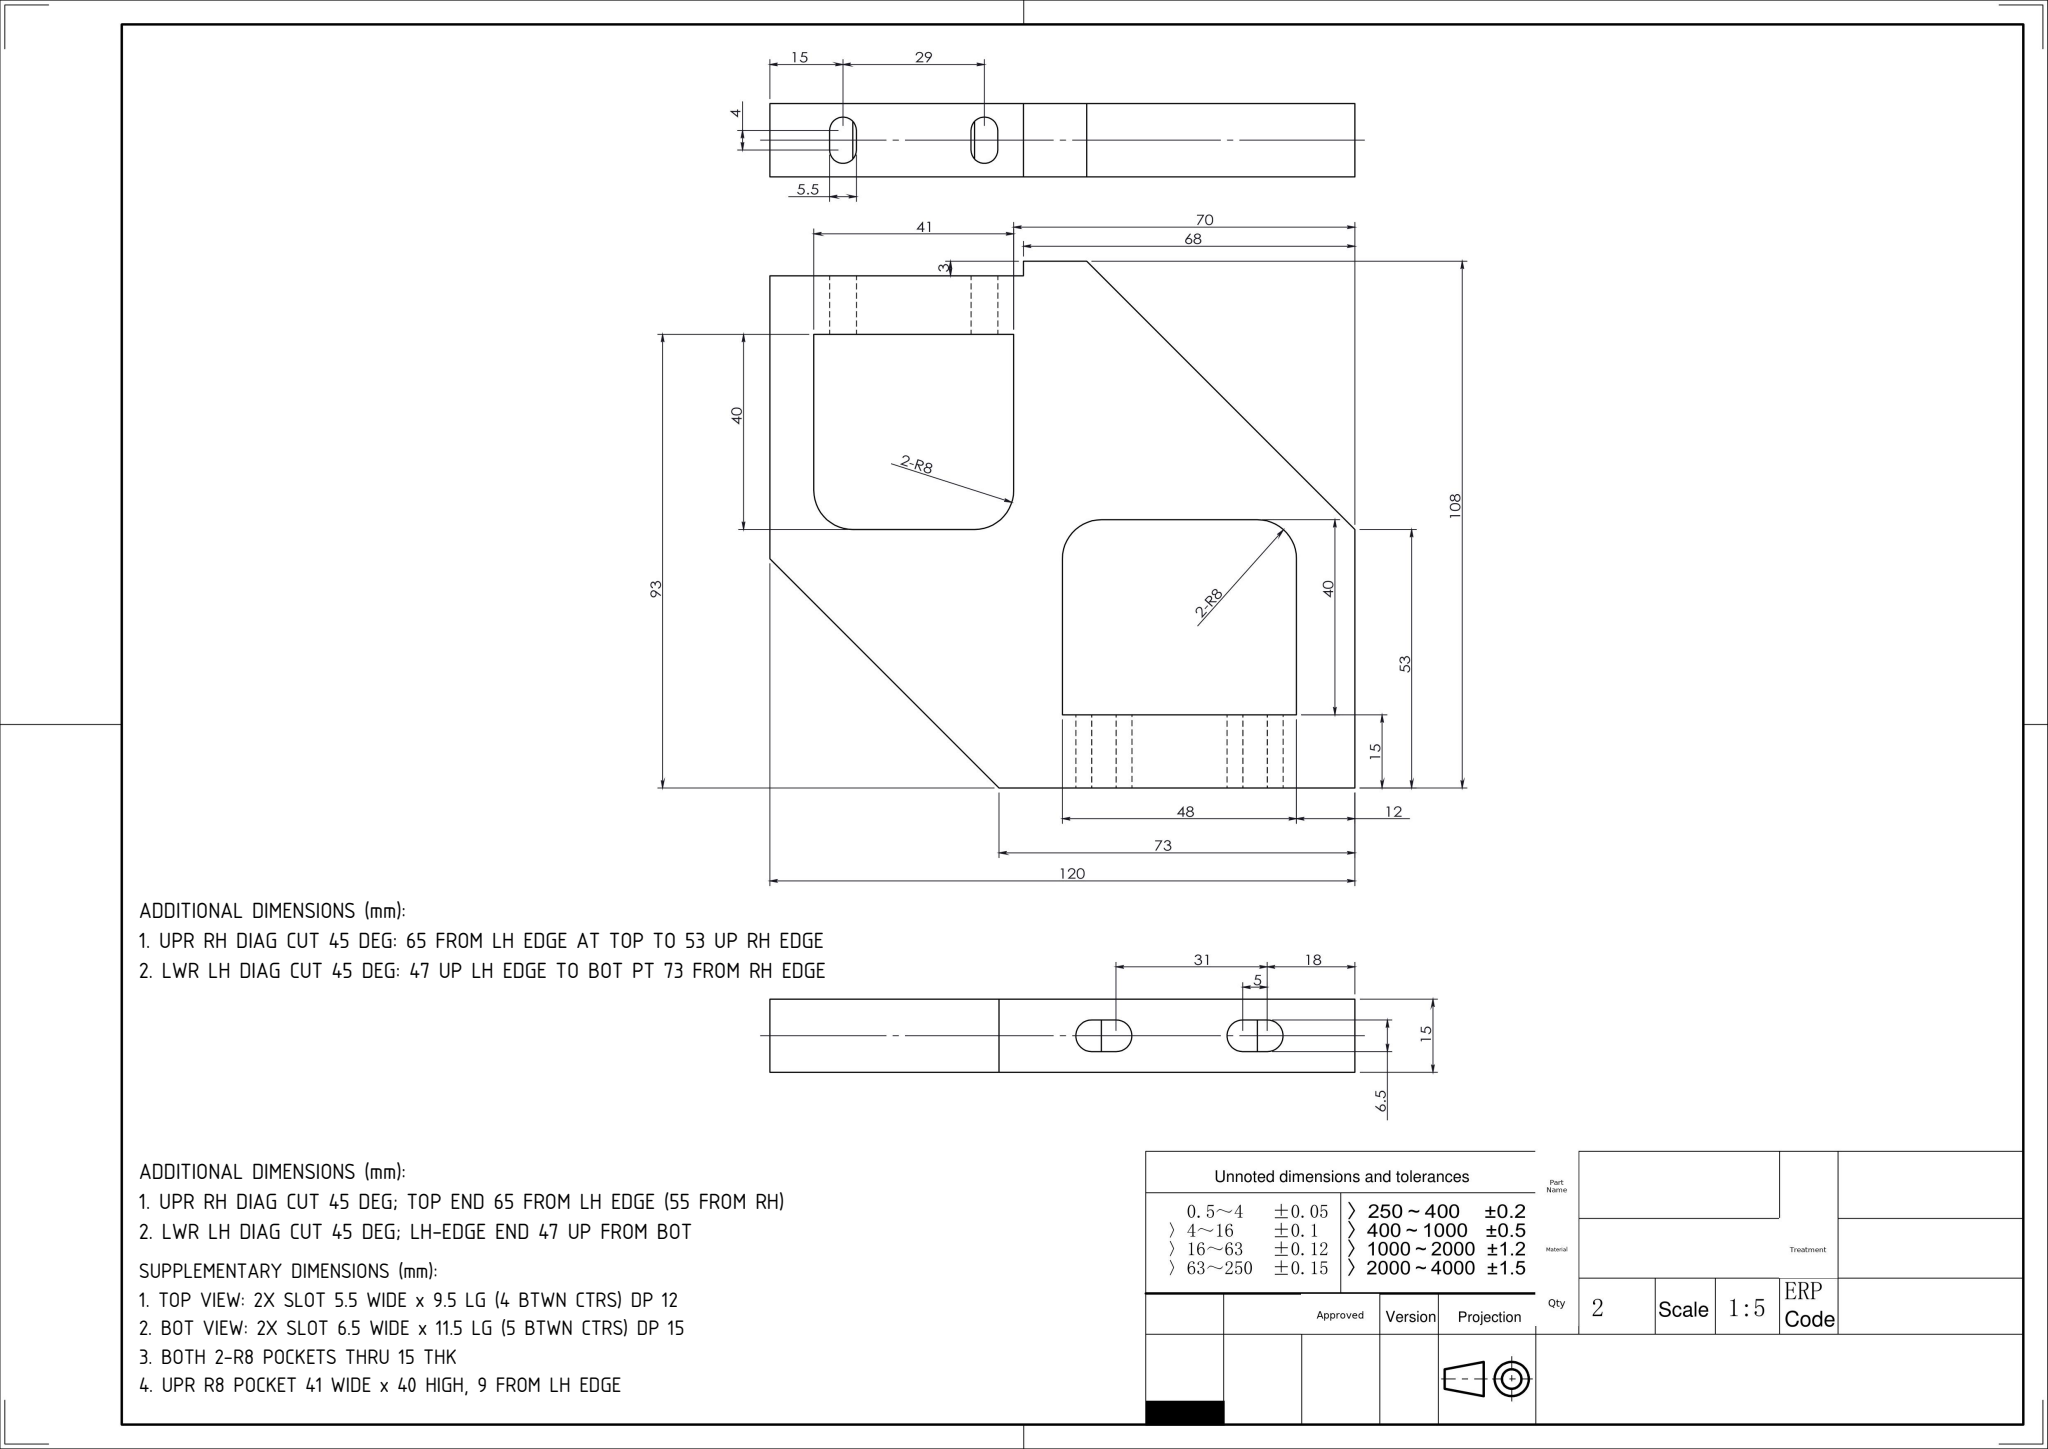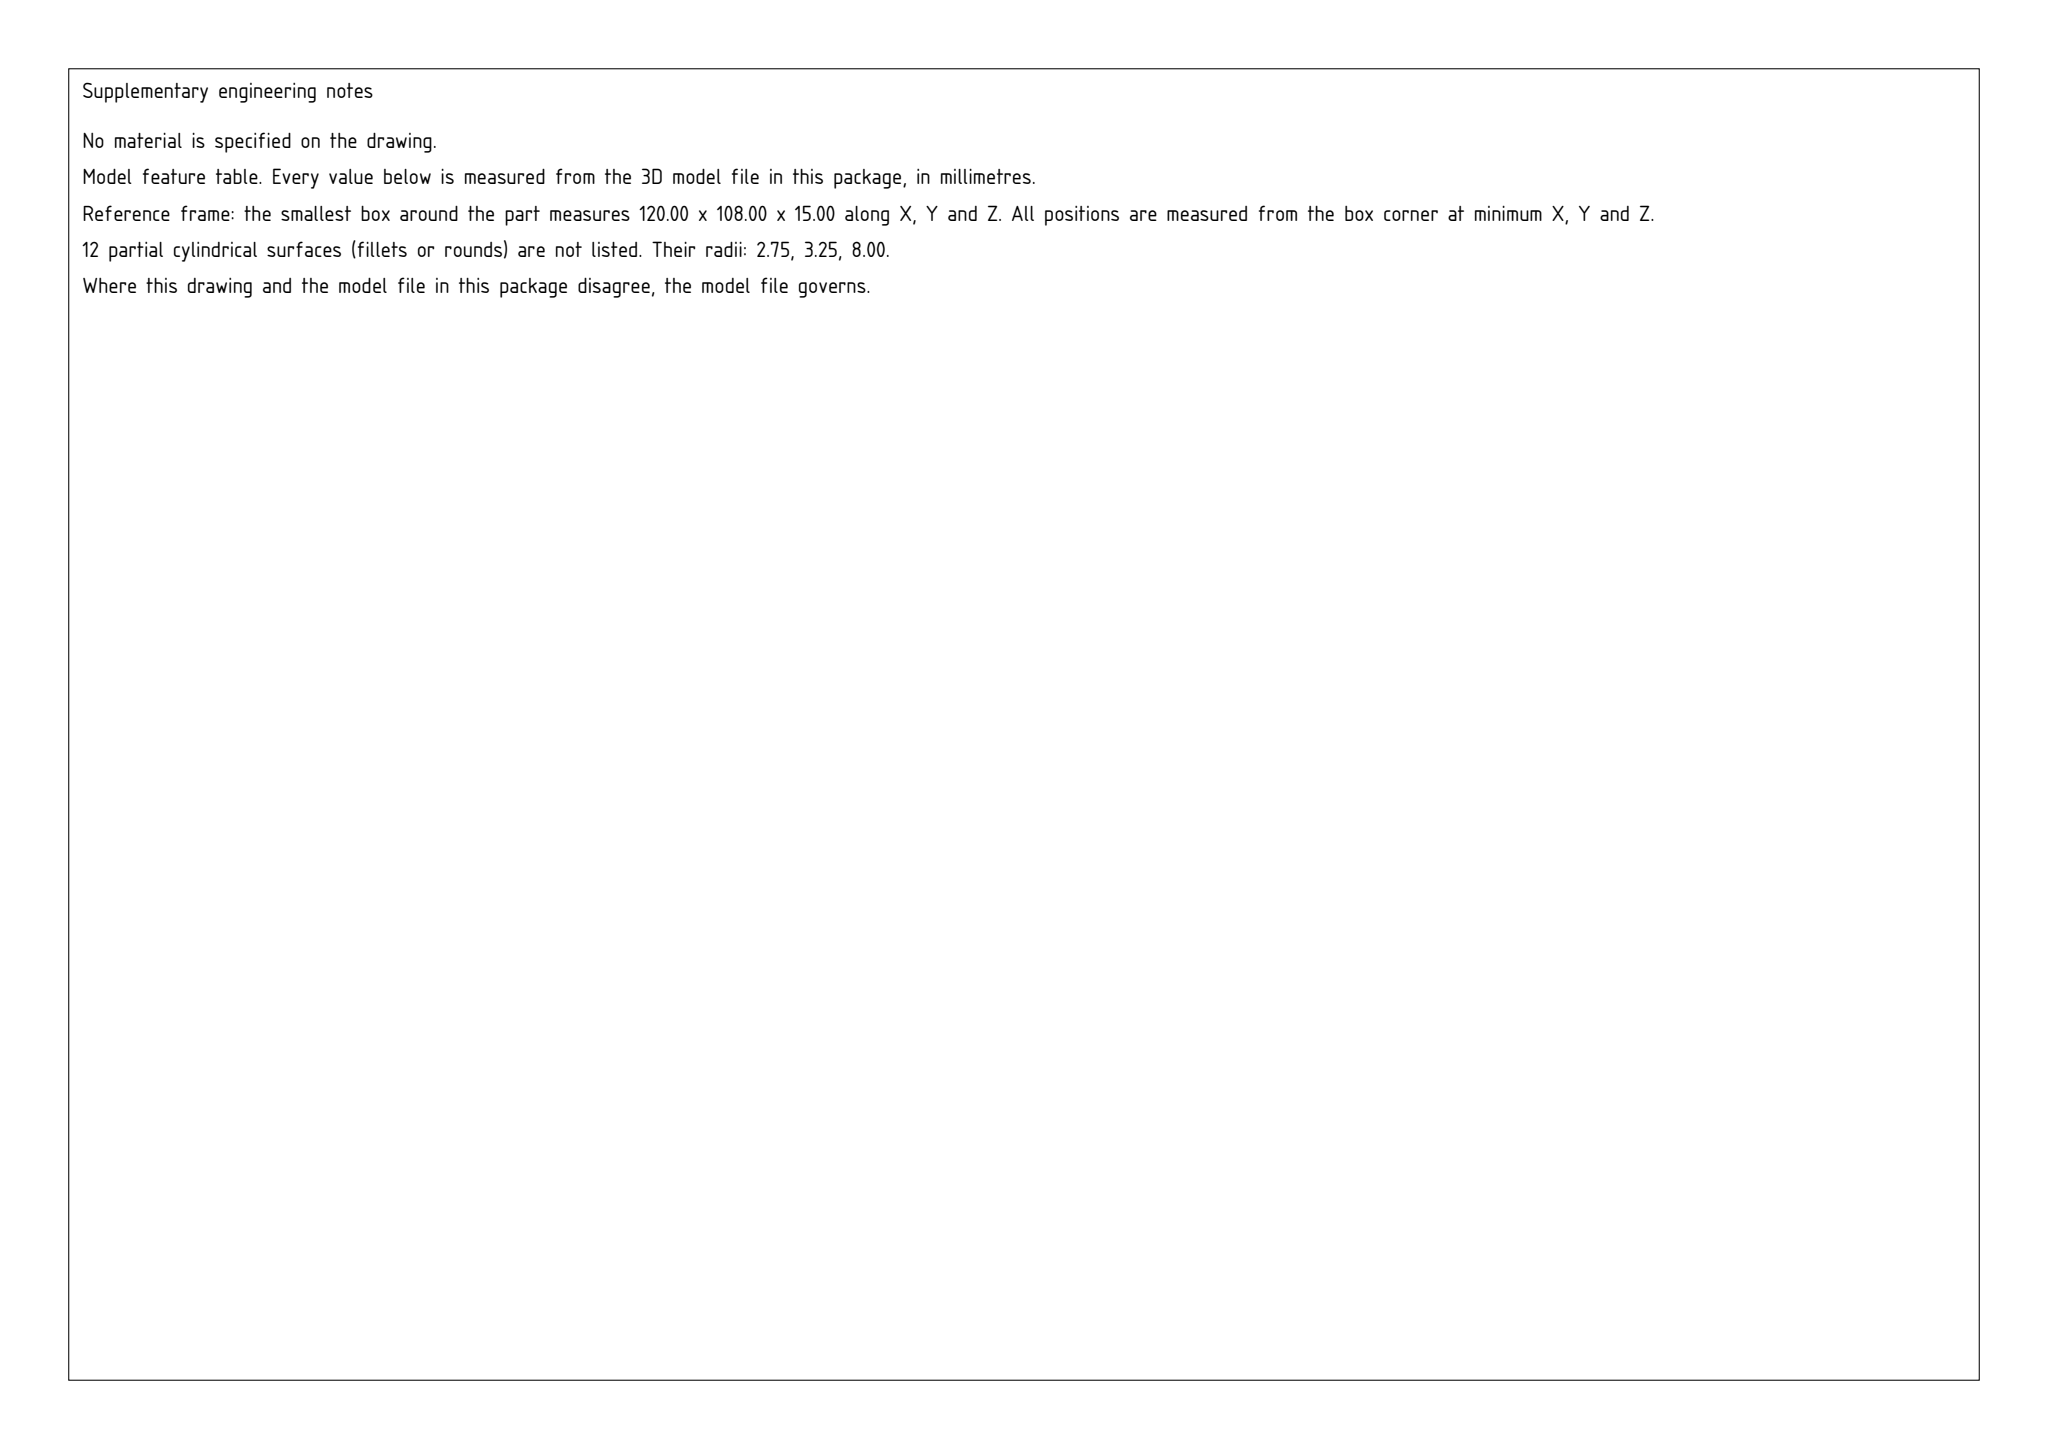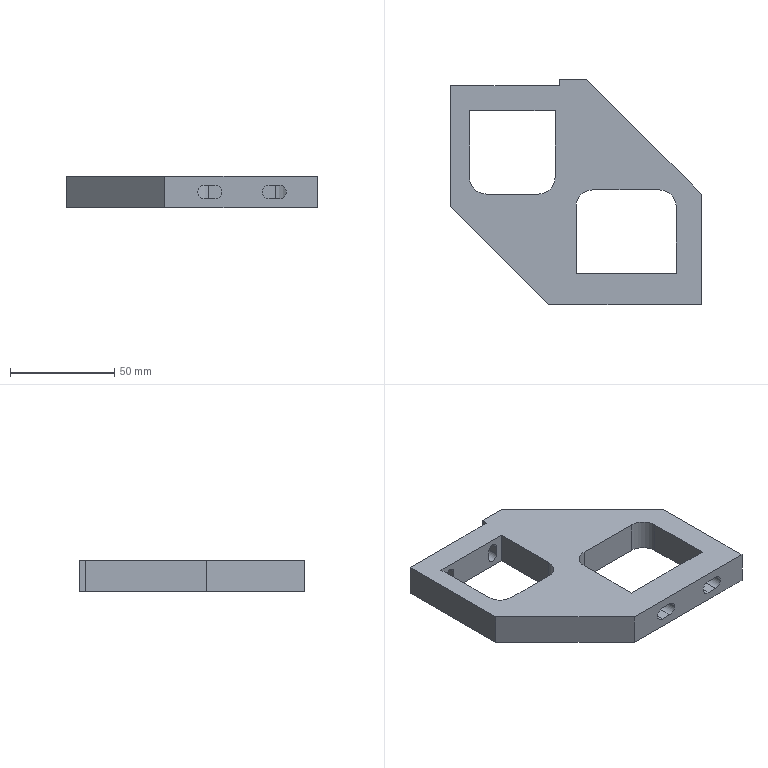Part | SolidWorks | mm | 1 solid | 42 faces | box 120 x 108 x 15 mm | volume 97160 mm3 | plane 26 | cylinder 16 | commonest cylinder face diameters 6.5 x6 5.5 x6 16 x4
build123d program:
from build123d import *

# Parameters (mm, degrees)
BOSS_EXTRUDE1_DEPTH   = 15
M5_TAPPED_HOLE2_D     = 4.2
M5_TAPPED_HOLE2_DEPTH = 14
M5_TAPPED_HOLE2_TIP   = 1.262
CUT_EXTRUDE2_DEPTH    = 25
SKETCH7_W             = 41
SKETCH7_H             = 40
SKETCH7_W_2           = 48
CUT_EXTRUDE1_DEPTH    = 163.139
SKETCH10_W            = 52
SKETCH10_H            = 15
CUT_EXTRUDE3_DEPTH    = 3
CUT_EXTRUDE4_DEPTH    = 20
FILLET1_R             = 8
CHAMFER1_SIZE         = 47


with BuildPart() as part:
    # Sketch1 → Boss-Extrude1 (new body)
    with BuildSketch(Plane.XY):
        Polygon((0, 0), (0, 108), (65, 108), (120, 53), (120, 0), align=None)
    extrude(amount=BOSS_EXTRUDE1_DEPTH)

    # M5 Tapped Hole2
    with Locations(Plane.XZ):
        with Locations((39, 10)):
            Hole(M5_TAPPED_HOLE2_D / 2, depth=M5_TAPPED_HOLE2_DEPTH)
            with Locations((0, 0, -(M5_TAPPED_HOLE2_DEPTH + M5_TAPPED_HOLE2_TIP / 2))):  # 118° drill point
                Cone(0, M5_TAPPED_HOLE2_D / 2, M5_TAPPED_HOLE2_TIP, mode=Mode.SUBTRACT)

    # Sketch8 → Cut-Extrude2 (cut)
    with BuildSketch(Plane(origin=(0, 108, 0), x_dir=(1, 0, 0), z_dir=(0, 1, 0))):
        with BuildLine():
            Line((17.75, -5.5), (17.75, -9.5))
            ThreePointArc((17.75, -9.5), (15, -12.25), (12.25, -9.5))
            Line((12.25, -9.5), (12.25, -5.5))
            ThreePointArc((12.25, -5.5), (15, -2.75), (17.75, -5.5))
        make_face()
        with BuildLine():
            Line((46.75, -5.5), (46.75, -9.5))
            ThreePointArc((46.75, -9.5), (44, -12.25), (41.25, -9.5))
            Line((41.25, -9.5), (41.25, -5.5))
            ThreePointArc((41.25, -5.5), (44, -2.75), (46.75, -5.5))
        make_face()
    extrude(amount=-CUT_EXTRUDE2_DEPTH, mode=Mode.SUBTRACT)

    # Sketch7 → Cut-Extrude1 (cut, through all)
    with BuildSketch(Plane.XY.offset(15)):
        with Locations((29.5, 73)):
            Rectangle(SKETCH7_W, SKETCH7_H)
        with Locations((84, 35)):
            Rectangle(SKETCH7_W_2, SKETCH7_H)
    extrude(amount=-CUT_EXTRUDE1_DEPTH, mode=Mode.SUBTRACT)

    # Sketch10 → Cut-Extrude3 (cut)
    with BuildSketch(Plane(origin=(0, 108, 0), x_dir=(1, 0, 0), z_dir=(0, 1, 0))):
        with Locations((26, -7.5)):
            Rectangle(SKETCH10_W, SKETCH10_H)
    extrude(amount=-CUT_EXTRUDE3_DEPTH, mode=Mode.SUBTRACT)

    # Sketch11 → Cut-Extrude4 (cut)
    with BuildSketch(Plane.XZ):
        with BuildLine():
            ThreePointArc((71, 4.25), (74.25, 7.5), (71, 10.75))
            Line((71, 10.75), (66, 10.75))
            ThreePointArc((66, 10.75), (62.75, 7.5), (66, 4.25))
            Line((66, 4.25), (71, 4.25))
        make_face()
        with BuildLine():
            ThreePointArc((102, 4.25), (105.25, 7.5), (102, 10.75))
            Line((102, 10.75), (97, 10.75))
            ThreePointArc((97, 10.75), (93.75, 7.5), (97, 4.25))
            Line((97, 4.25), (102, 4.25))
        make_face()
    extrude(amount=-CUT_EXTRUDE4_DEPTH, mode=Mode.SUBTRACT)

    # Fillet1
    fillet1_edges = [part.edges().sort_by_distance(p)[0] for p in [
        (9, 53, 7.5),
        (50, 53, 7.5),
        (60, 55, 7.5),
        (108, 55, 7.5),
    ]]
    fillet(fillet1_edges, radius=FILLET1_R)

    # Chamfer1
    chamfer1_edges = [part.edges().sort_by_distance(p)[0] for p in [
        (0, 0, 7.5),
    ]]
    chamfer(chamfer1_edges, length=CHAMFER1_SIZE)


solid = part.part